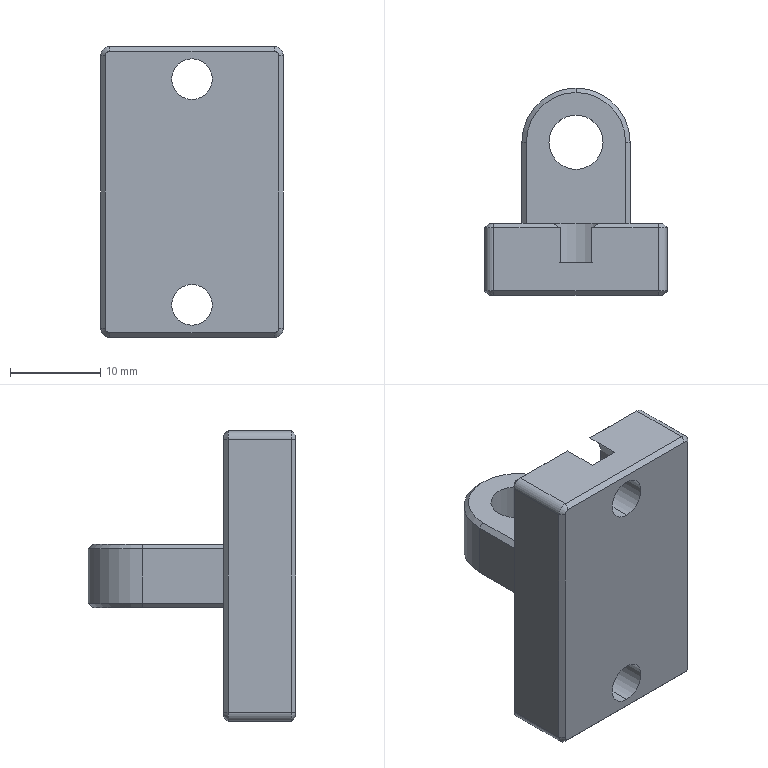Part | SolidWorks | mm | 1 solid | 53 faces | box 20.2 x 23 x 32.2 mm | volume 5568 mm3 | plane 26 | cylinder 15 | cone 12 | commonest cylinder face diameters 4.5 x4 2 x4 8 x3 6 x2 12 x2